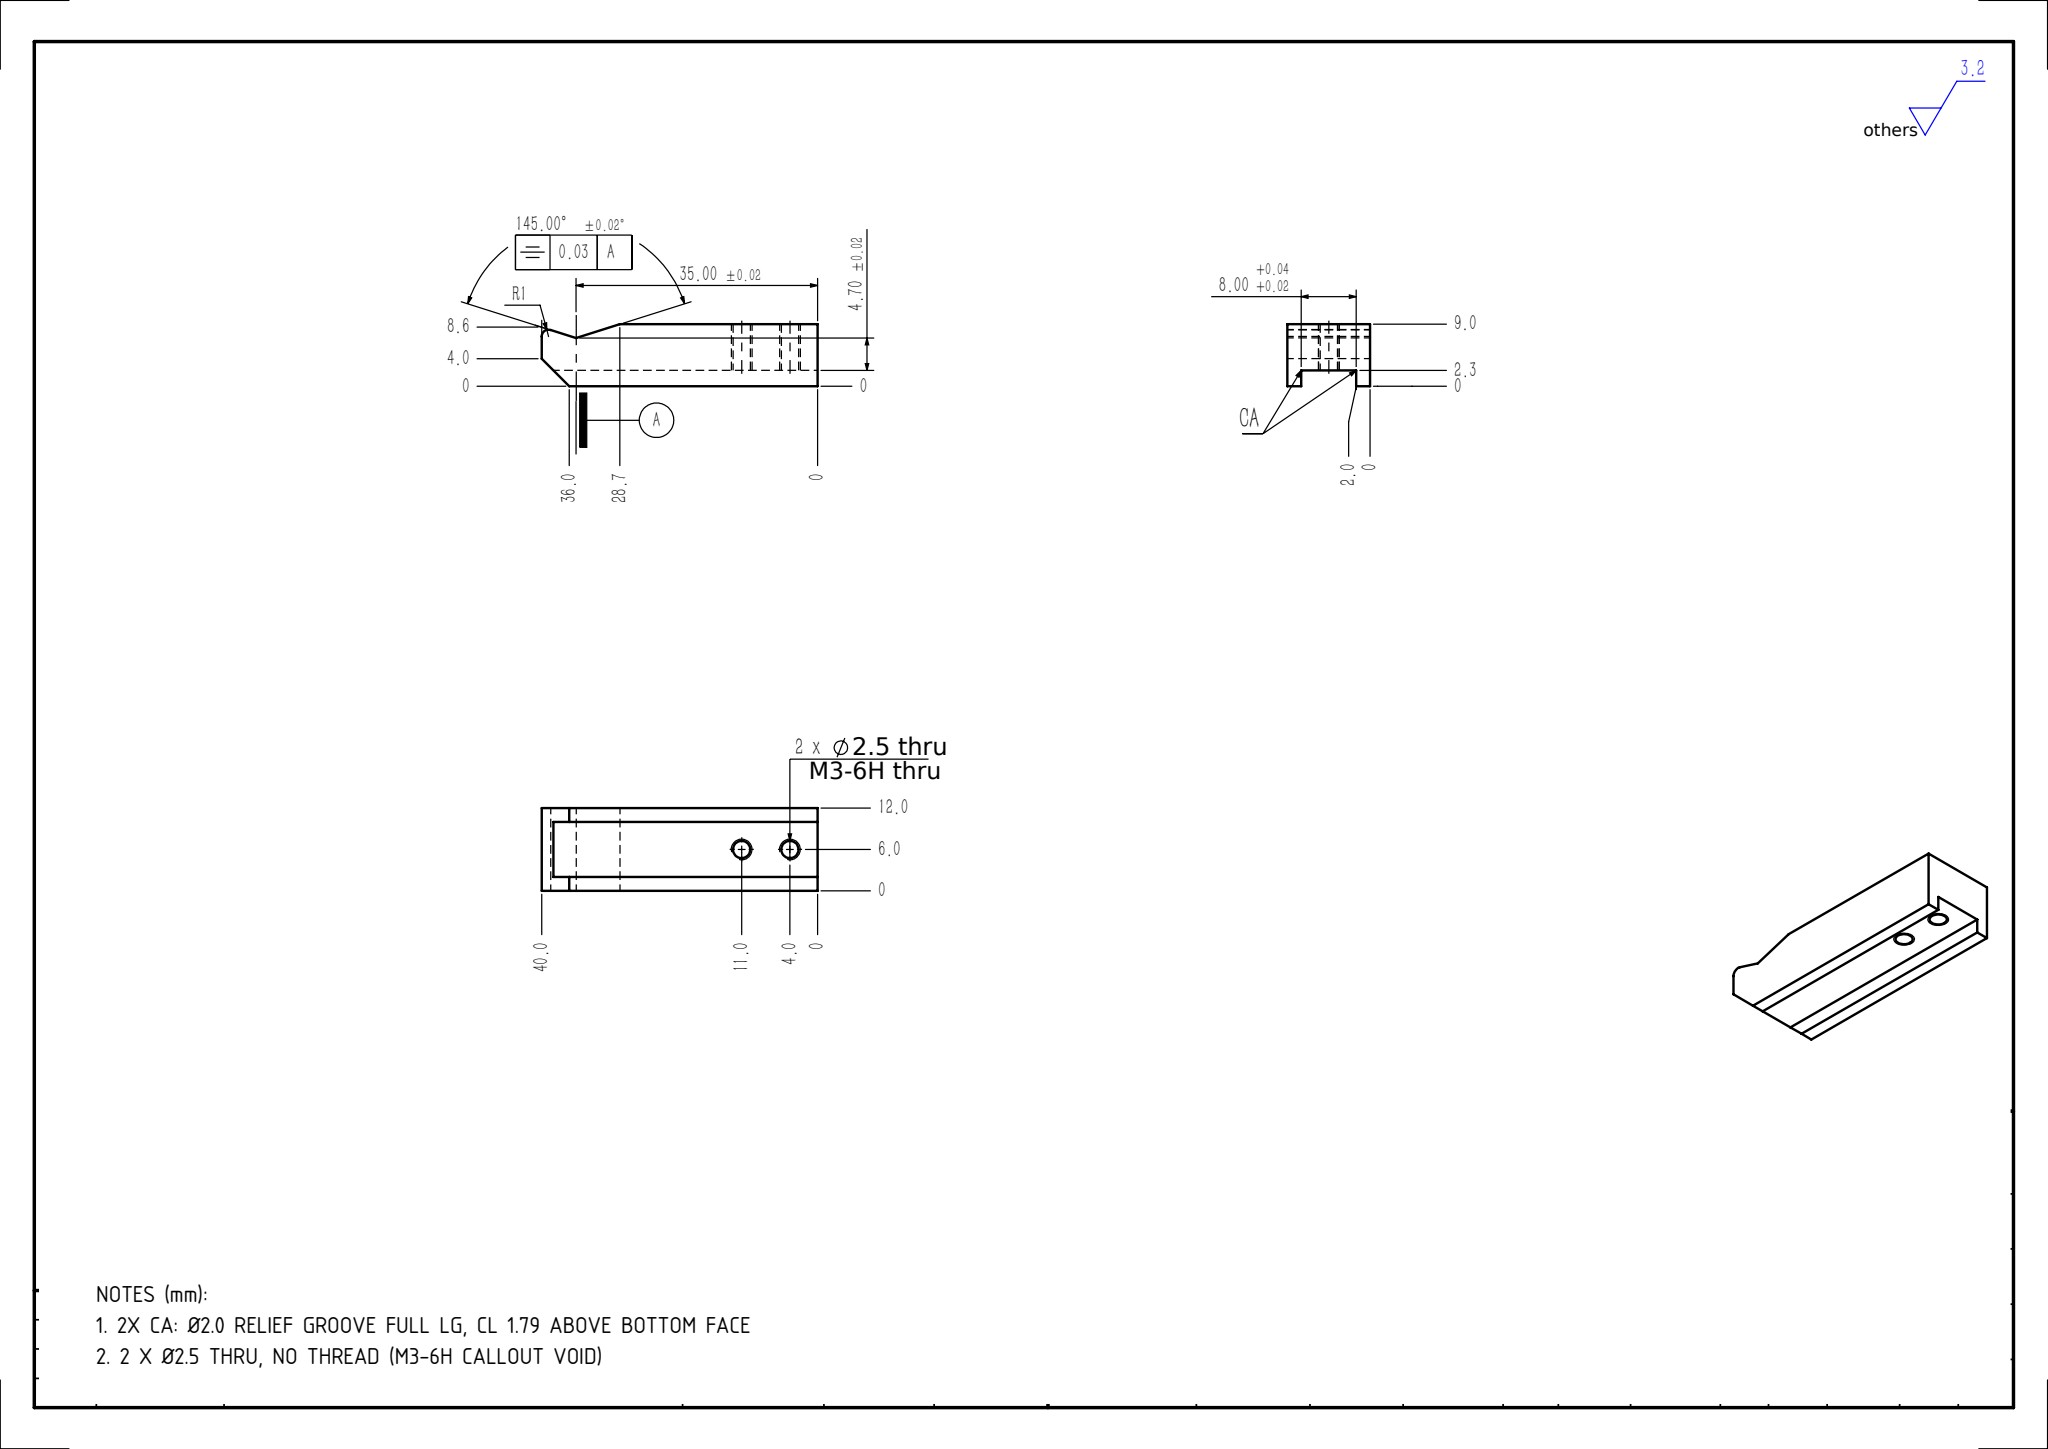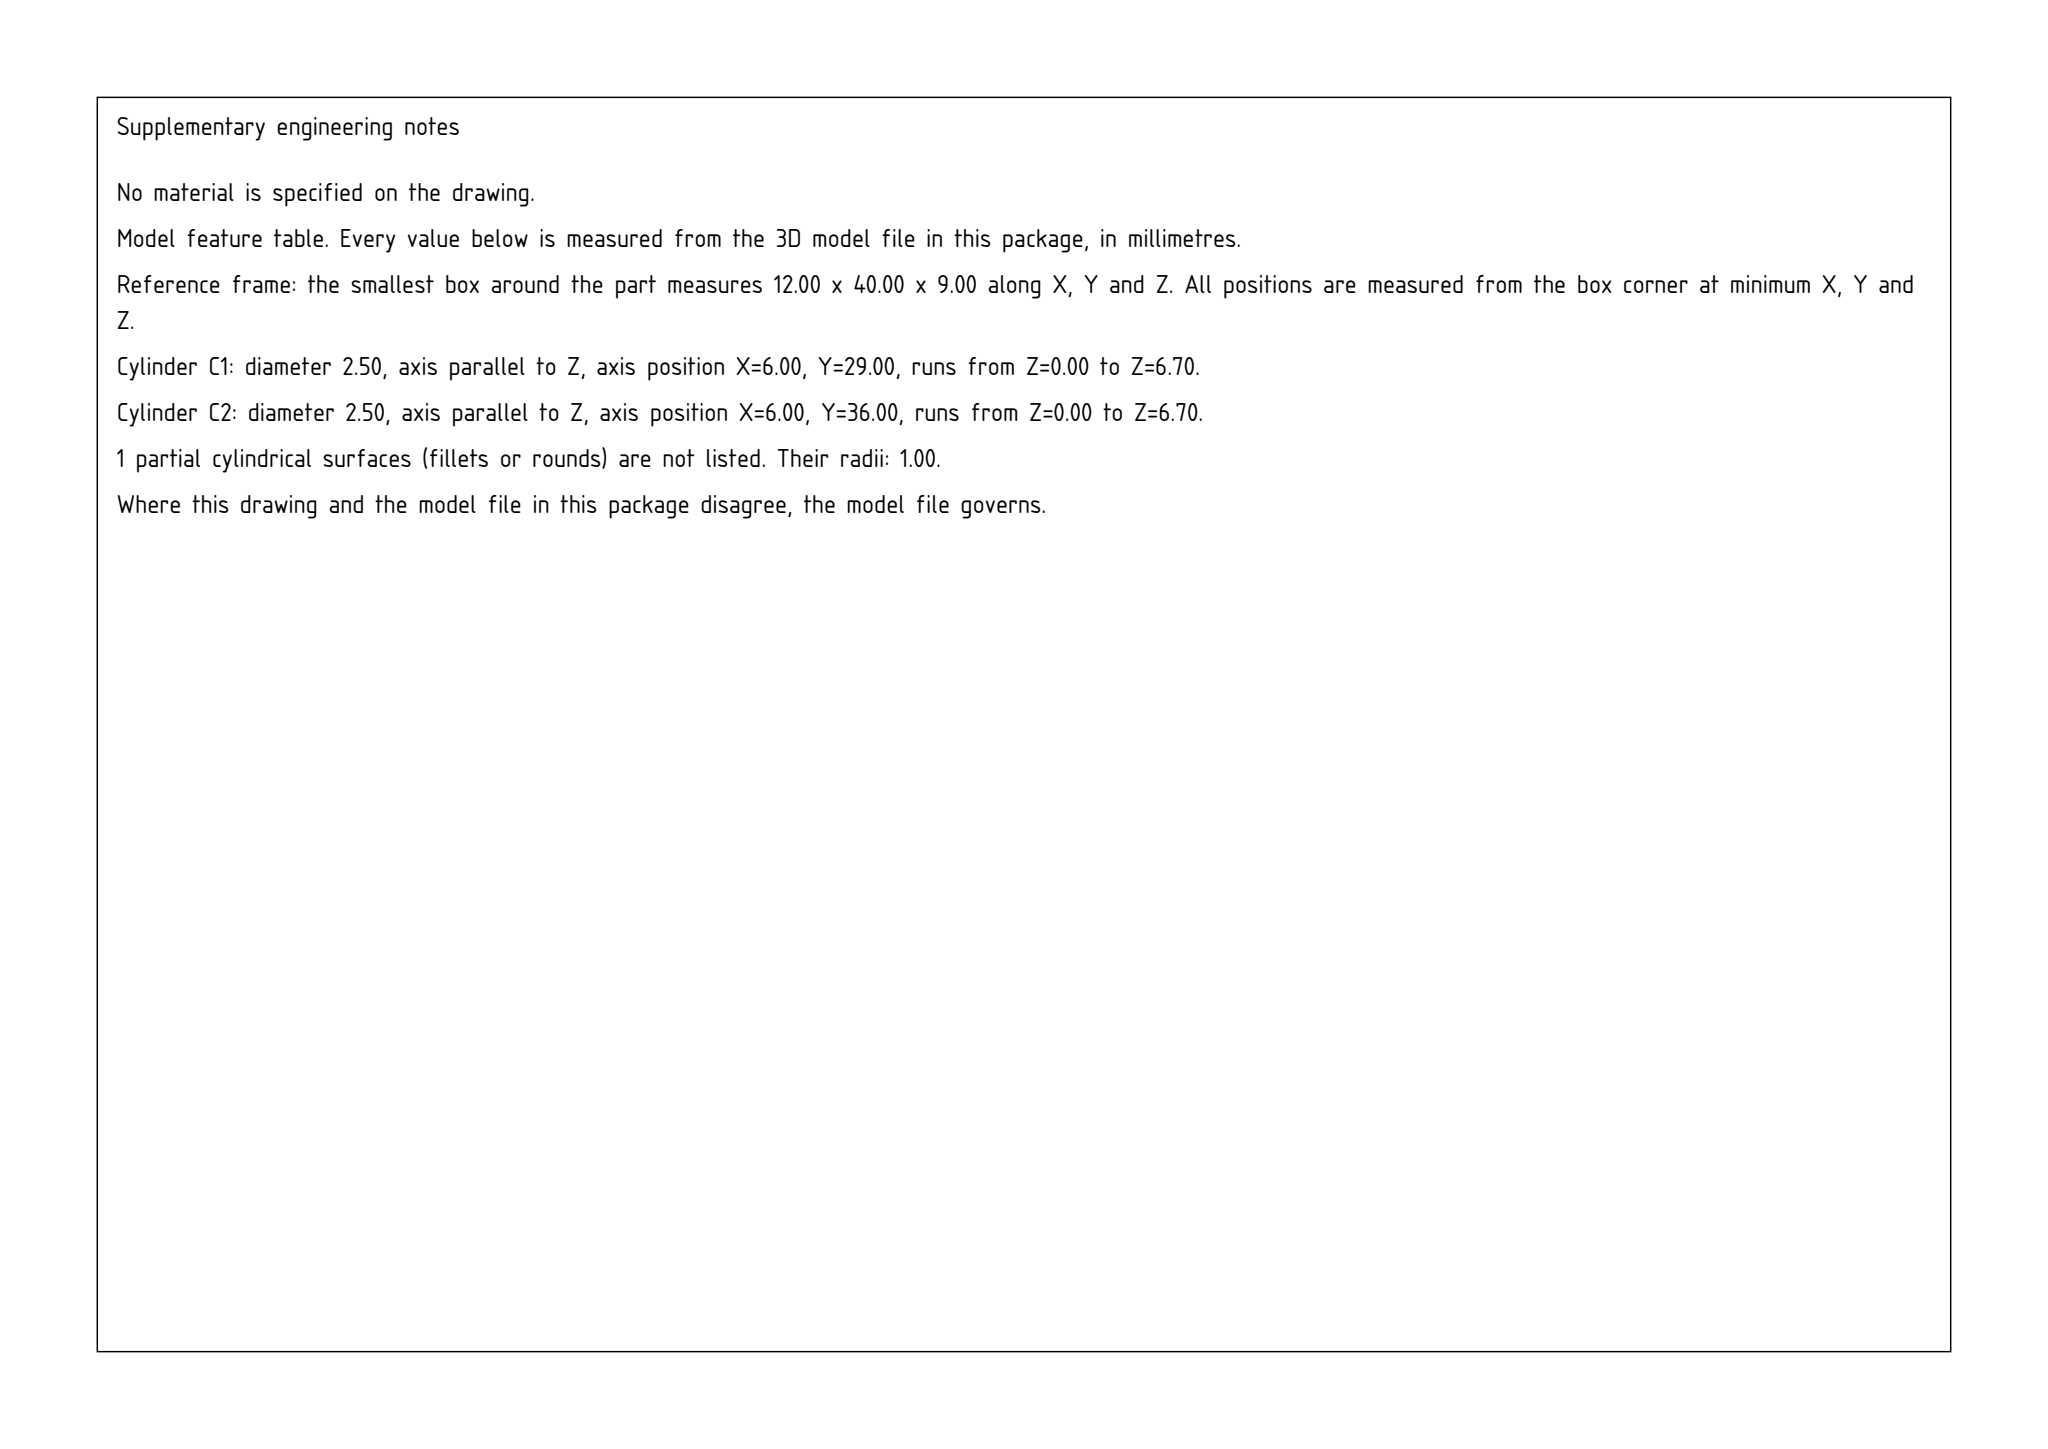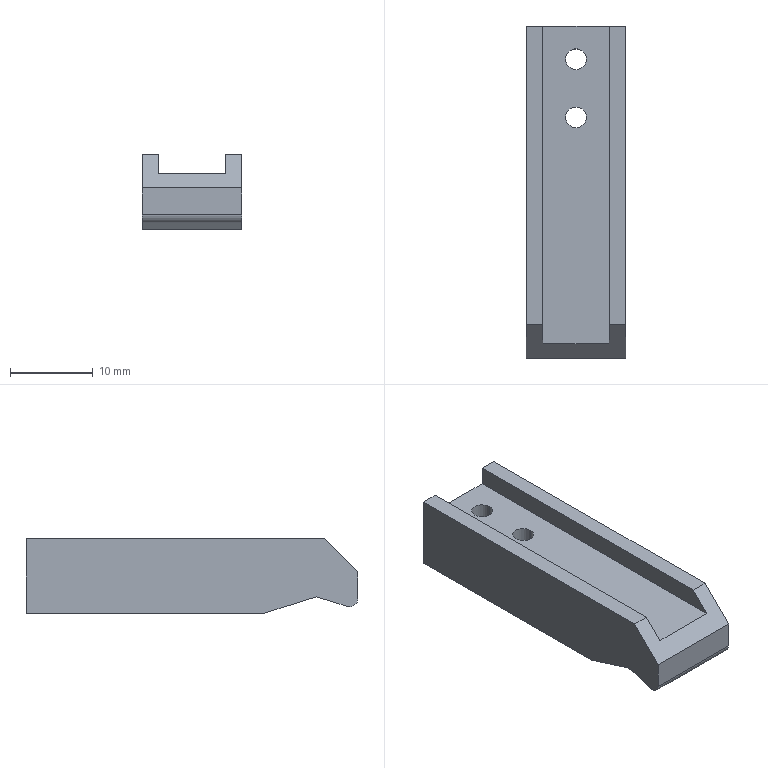Part | SolidWorks | mm | 1 solid | 19 faces | box 12 x 40 x 9 mm | volume 3321 mm3 | plane 13 | cylinder 6 | commonest cylinder face diameters 2.5 x4 2 x2
Drawing notes:
2X CA: Ø2.0 RELIEF GROOVE FULL LG, CL 1.79 ABOVE BOTTOM FACE | from the solid: cylinders [2.0,"x",[null,1.0,1.79],12.0,2] - Ø2.0 grooves, full length, axis 1.79 above z=0 base, at inner corners of 8.00 channel (x=2.0 & x=10.0 walls, floor z=2.3)
2 X Ø2.5 THRU, NO THREAD (M3-6H CALLOUT VOID) | from the solid: cylinders dia 2.5 along z at (x=6.0, y=29.0) and (x=6.0, y=36.0), length 6.7 = full 6.7 wall thickness (z planes 0 and 6.7); no thread/cone features in STEP
STEP:
#1=CARTESIAN_POINT('',(0.,-39.,0.7873));
#2=VERTEX_POINT('',#1);
#3=CARTESIAN_POINT('',(0.,-40.,1.787));
#4=VERTEX_POINT('',#3);
#5=CARTESIAN_POINT('',(0.,-39.,1.787));
#6=DIRECTION('',(-1.,-0.,0.));
#7=DIRECTION('',(-0.,1.,0.));
#8=AXIS2_PLACEMENT_3D('',#5,#6,#7);
#9=CIRCLE('',#8,1.);
#10=EDGE_CURVE('',#2,#4,#9,.T.);
#11=ORIENTED_EDGE('',*,*,#10,.F.);
#12=CARTESIAN_POINT('',(12.,-39.,0.7873));
#13=VERTEX_POINT('',#12);
#14=CARTESIAN_POINT('',(0.,-39.,0.7873));
#15=DIRECTION('',(1.,0.,-0.));
#16=VECTOR('',#15,1000.);
#17=LINE('',#14,#16);
#18=EDGE_CURVE('',#2,#13,#17,.T.);
#19=ORIENTED_EDGE('',*,*,#18,.T.);
#20=CARTESIAN_POINT('',(12.,-40.,1.787));
#21=VERTEX_POINT('',#20);
#22=CARTESIAN_POINT('',(12.,-39.,1.787));
#23=DIRECTION('',(1.,0.,0.));
#24=DIRECTION('',(0.,-1.,0.));
#25=AXIS2_PLACEMENT_3D('',#22,#23,#24);
#26=CIRCLE('',#25,1.);
#27=EDGE_CURVE('',#21,#13,#26,.T.);
#28=ORIENTED_EDGE('',*,*,#27,.F.);
#29=CARTESIAN_POINT('',(0.,-40.,1.787));
#30=DIRECTION('',(1.,0.,-0.));
#31=VECTOR('',#30,1000.);
#32=LINE('',#29,#31);
#33=EDGE_CURVE('',#4,#21,#32,.T.);
#34=ORIENTED_EDGE('',*,*,#33,.F.);
#35=EDGE_LOOP('',(#11,#19,#28,#34));
#36=FACE_OUTER_BOUND('',#35,.T.);
#37=CARTESIAN_POINT('',(0.,-39.,1.787));
#38=DIRECTION('',(1.,0.,-0.));
#39=DIRECTION('',(-0.,0.,-1.));
#40=AXIS2_PLACEMENT_3D('',#37,#38,#39);
#41=CYLINDRICAL_SURFACE('',#40,1.);
#42=ADVANCED_FACE('',(#36),#41,.T.);
#43=CARTESIAN_POINT('',(4.75,-4.,0.));
#44=VERTEX_POINT('',#43);
#45=CARTESIAN_POINT('',(7.25,-4.,0.));
#46=VERTEX_POINT('',#45);
#47=CARTESIAN_POINT('',(6.,-4.,0.));
#48=DIRECTION('',(0.,0.,1.));
#49=DIRECTION('',(1.,0.,0.));
#50=AXIS2_PLACEMENT_3D('',#47,#48,#49);
#51=CIRCLE('',#50,1.25);
#52=EDGE_CURVE('',#44,#46,#51,.T.);
#53=ORIENTED_EDGE('',*,*,#52,.F.);
#54=CARTESIAN_POINT('',(4.75,-4.,6.7));
#55=VERTEX_POINT('',#54);
#56=CARTESIAN_POINT('',(4.75,-4.,6.7));
#57=DIRECTION('',(0.,0.,1.));
#58=VECTOR('',#57,1000.);
#59=LINE('',#56,#58);
#60=EDGE_CURVE('',#44,#55,#59,.T.);
#61=ORIENTED_EDGE('',*,*,#60,.T.);
#62=CARTESIAN_POINT('',(7.25,-4.,6.7));
#63=VERTEX_POINT('',#62);
#64=CARTESIAN_POINT('',(6.,-4.,6.7));
#65=DIRECTION('',(0.,0.,1.));
#66=DIRECTION('',(1.,0.,0.));
#67=AXIS2_PLACEMENT_3D('',#64,#65,#66);
#68=CIRCLE('',#67,1.25);
#69=EDGE_CURVE('',#55,#63,#68,.T.);
#70=ORIENTED_EDGE('',*,*,#69,.T.);
#71=CARTESIAN_POINT('',(7.25,-4.,6.7));
#72=DIRECTION('',(0.,0.,1.));
#73=VECTOR('',#72,1000.);
#74=LINE('',#71,#73);
#75=EDGE_CURVE('',#46,#63,#74,.T.);
#76=ORIENTED_EDGE('',*,*,#75,.F.);
#77=EDGE_LOOP('',(#53,#61,#70,#76));
#78=FACE_OUTER_BOUND('',#77,.T.);
#79=CARTESIAN_POINT('',(6.,-4.,6.7));
#80=DIRECTION('',(0.,0.,1.));
#81=DIRECTION('',(1.,0.,0.));
#82=AXIS2_PLACEMENT_3D('',#79,#80,#81);
#83=CYLINDRICAL_SURFACE('',#82,1.25);
#84=ADVANCED_FACE('',(#78),#83,.F.);
#85=CARTESIAN_POINT('',(4.75,-11.,0.));
#86=VERTEX_POINT('',#85);
#87=CARTESIAN_POINT('',(7.25,-11.,0.));
#88=VERTEX_POINT('',#87);
#89=CARTESIAN_POINT('',(6.,-11.,0.));
#90=DIRECTION('',(0.,0.,1.));
#91=DIRECTION('',(1.,0.,0.));
#92=AXIS2_PLACEMENT_3D('',#89,#90,#91);
#93=CIRCLE('',#92,1.25);
#94=EDGE_CURVE('',#86,#88,#93,.T.);
#95=ORIENTED_EDGE('',*,*,#94,.F.);
#96=CARTESIAN_POINT('',(4.75,-11.,6.7));
#97=VERTEX_POINT('',#96);
#98=CARTESIAN_POINT('',(4.75,-11.,6.7));
#99=DIRECTION('',(0.,0.,1.));
#100=VECTOR('',#99,1000.);
#101=LINE('',#98,#100);
#102=EDGE_CURVE('',#86,#97,#101,.T.);
#103=ORIENTED_EDGE('',*,*,#102,.T.);
#104=CARTESIAN_POINT('',(7.25,-11.,6.7));
#105=VERTEX_POINT('',#104);
#106=CARTESIAN_POINT('',(6.,-11.,6.7));
#107=DIRECTION('',(0.,0.,1.));
#108=DIRECTION('',(1.,0.,0.));
#109=AXIS2_PLACEMENT_3D('',#106,#107,#108);
#110=CIRCLE('',#109,1.25);
#111=EDGE_CURVE('',#97,#105,#110,.T.);
#112=ORIENTED_EDGE('',*,*,#111,.T.);
#113=CARTESIAN_POINT('',(7.25,-11.,6.7));
#114=DIRECTION('',(0.,0.,1.));
#115=VECTOR('',#114,1000.);
#116=LINE('',#113,#115);
#117=EDGE_CURVE('',#88,#105,#116,.T.);
#118=ORIENTED_EDGE('',*,*,#117,.F.);
#119=EDGE_LOOP('',(#95,#103,#112,#118));
#120=FACE_OUTER_BOUND('',#119,.T.);
#121=CARTESIAN_POINT('',(6.,-11.,6.7));
#122=DIRECTION('',(0.,0.,1.));
#123=DIRECTION('',(1.,0.,0.));
#124=AXIS2_PLACEMENT_3D('',#121,#122,#123);
#125=CYLINDRICAL_SURFACE('',#124,1.25);
#126=ADVANCED_FACE('',(#120),#125,.F.);
#127=CARTESIAN_POINT('',(0.,0.,9.));
#128=VERTEX_POINT('',#127);
#129=CARTESIAN_POINT('',(0.,-36.,9.));
#130=VERTEX_POINT('',#129);
#131=CARTESIAN_POINT('',(0.,0.,9.));
#132=DIRECTION('',(0.,-1.,0.));
#133=VECTOR('',#132,1000.);
#134=LINE('',#131,#133);
#135=EDGE_CURVE('',#128,#130,#134,.T.);
#136=ORIENTED_EDGE('',*,*,#135,.T.);
#137=CARTESIAN_POINT('',(2.,-36.,9.));
#138=VERTEX_POINT('',#137);
#139=CARTESIAN_POINT('',(2.,-36.,9.));
#140=DIRECTION('',(1.,0.,0.));
#141=VECTOR('',#140,1000.);
#142=LINE('',#139,#141);
#143=EDGE_CURVE('',#130,#138,#142,.T.);
#144=ORIENTED_EDGE('',*,*,#143,.T.);
#145=CARTESIAN_POINT('',(2.,-0.,9.));
#146=VERTEX_POINT('',#145);
#147=CARTESIAN_POINT('',(2.,-0.,9.));
#148=DIRECTION('',(0.,-1.,0.));
#149=VECTOR('',#148,1000.);
#150=LINE('',#147,#149);
#151=EDGE_CURVE('',#146,#138,#150,.T.);
#152=ORIENTED_EDGE('',*,*,#151,.F.);
#153=CARTESIAN_POINT('',(0.,0.,9.));
#154=DIRECTION('',(-1.,0.,0.));
#155=VECTOR('',#154,1000.);
#156=LINE('',#153,#155);
#157=EDGE_CURVE('',#146,#128,#156,.T.);
#158=ORIENTED_EDGE('',*,*,#157,.T.);
#159=EDGE_LOOP('',(#136,#144,#152,#158));
#160=FACE_OUTER_BOUND('',#159,.T.);
#161=CARTESIAN_POINT('',(0.,0.,9.));
#162=DIRECTION('',(0.,0.,1.));
#163=DIRECTION('',(1.,0.,0.));
#164=AXIS2_PLACEMENT_3D('',#161,#162,#163);
#165=PLANE('',#164);
#166=ADVANCED_FACE('',(#160),#165,.T.);
#167=CARTESIAN_POINT('',(0.,-35.,2.));
#168=VERTEX_POINT('',#167);
#169=CARTESIAN_POINT('',(0.,-38.699,0.8336));
#170=VERTEX_POINT('',#169);
#171=CARTESIAN_POINT('',(0.,-35.,2.));
#172=DIRECTION('',(0.,-0.9537,-0.3007));
#173=VECTOR('',#172,1000.);
#174=LINE('',#171,#173);
#175=EDGE_CURVE('',#168,#170,#174,.T.);
#176=ORIENTED_EDGE('',*,*,#175,.T.);
#177=CARTESIAN_POINT('',(0.,-39.,1.787));
#178=DIRECTION('',(-1.,-0.,0.));
#179=DIRECTION('',(-0.,1.,0.));
#180=AXIS2_PLACEMENT_3D('',#177,#178,#179);
#181=CIRCLE('',#180,1.);
#182=EDGE_CURVE('',#170,#2,#181,.T.);
#183=ORIENTED_EDGE('',*,*,#182,.T.);
#184=ORIENTED_EDGE('',*,*,#10,.T.);
#185=CARTESIAN_POINT('',(0.,-40.,5.));
#186=VERTEX_POINT('',#185);
#187=CARTESIAN_POINT('',(0.,-40.,9.));
#188=DIRECTION('',(0.,0.,-1.));
#189=VECTOR('',#188,1000.);
#190=LINE('',#187,#189);
#191=EDGE_CURVE('',#186,#4,#190,.T.);
#192=ORIENTED_EDGE('',*,*,#191,.F.);
#193=CARTESIAN_POINT('',(0.,-36.,9.));
#194=DIRECTION('',(-0.,0.7071,0.7071));
#195=VECTOR('',#194,1000.);
#196=LINE('',#193,#195);
#197=EDGE_CURVE('',#186,#130,#196,.T.);
#198=ORIENTED_EDGE('',*,*,#197,.T.);
#199=ORIENTED_EDGE('',*,*,#135,.F.);
#200=CARTESIAN_POINT('',(0.,0.,0.));
#201=VERTEX_POINT('',#200);
#202=CARTESIAN_POINT('',(0.,0.,9.));
#203=DIRECTION('',(0.,0.,-1.));
#204=VECTOR('',#203,1000.);
#205=LINE('',#202,#204);
#206=EDGE_CURVE('',#128,#201,#205,.T.);
#207=ORIENTED_EDGE('',*,*,#206,.T.);
#208=CARTESIAN_POINT('',(0.,-28.657,0.));
#209=VERTEX_POINT('',#208);
#210=CARTESIAN_POINT('',(0.,0.,0.));
#211=DIRECTION('',(0.,-1.,0.));
#212=VECTOR('',#211,1000.);
#213=LINE('',#210,#212);
#214=EDGE_CURVE('',#201,#209,#213,.T.);
#215=ORIENTED_EDGE('',*,*,#214,.T.);
#216=CARTESIAN_POINT('',(0.,-28.657,-0.));
#217=DIRECTION('',(0.,-0.9537,0.3007));
#218=VECTOR('',#217,1000.);
#219=LINE('',#216,#218);
#220=EDGE_CURVE('',#209,#168,#219,.T.);
#221=ORIENTED_EDGE('',*,*,#220,.T.);
#222=EDGE_LOOP('',(#176,#183,#184,#192,#198,#199,#207,#215,#221));
#223=FACE_OUTER_BOUND('',#222,.T.);
#224=CARTESIAN_POINT('',(0.,0.,9.));
#225=DIRECTION('',(1.,0.,0.));
#226=DIRECTION('',(-0.,1.,0.));
#227=AXIS2_PLACEMENT_3D('',#224,#225,#226);
#228=PLANE('',#227);
#229=ADVANCED_FACE('',(#223),#228,.F.);
#230=ORIENTED_EDGE('',*,*,#191,.T.);
#231=ORIENTED_EDGE('',*,*,#33,.T.);
#232=CARTESIAN_POINT('',(12.,-40.,5.));
#233=VERTEX_POINT('',#232);
#234=CARTESIAN_POINT('',(12.,-40.,9.));
#235=DIRECTION('',(0.,0.,-1.));
#236=VECTOR('',#235,1000.);
#237=LINE('',#234,#236);
#238=EDGE_CURVE('',#233,#21,#237,.T.);
#239=ORIENTED_EDGE('',*,*,#238,.F.);
#240=CARTESIAN_POINT('',(10.,-40.,5.));
#241=DIRECTION('',(-1.,0.,0.));
#242=VECTOR('',#241,1000.);
#243=LINE('',#240,#242);
#244=EDGE_CURVE('',#233,#186,#243,.T.);
#245=ORIENTED_EDGE('',*,*,#244,.T.);
#246=EDGE_LOOP('',(#230,#231,#239,#245));
#247=FACE_OUTER_BOUND('',#246,.T.);
#248=CARTESIAN_POINT('',(0.,-40.,9.));
#249=DIRECTION('',(0.,1.,0.));
#250=DIRECTION('',(0.,0.,1.));
#251=AXIS2_PLACEMENT_3D('',#248,#249,#250);
#252=PLANE('',#251);
#253=ADVANCED_FACE('',(#247),#252,.F.);
#254=ORIENTED_EDGE('',*,*,#238,.T.);
#255=ORIENTED_EDGE('',*,*,#27,.T.);
#256=CARTESIAN_POINT('',(12.,-38.699,0.8336));
#257=VERTEX_POINT('',#256);
#258=CARTESIAN_POINT('',(12.,-39.,1.787));
#259=DIRECTION('',(1.,0.,0.));
#260=DIRECTION('',(0.,-1.,0.));
#261=AXIS2_PLACEMENT_3D('',#258,#259,#260);
#262=CIRCLE('',#261,1.);
#263=EDGE_CURVE('',#13,#257,#262,.T.);
#264=ORIENTED_EDGE('',*,*,#263,.T.);
#265=CARTESIAN_POINT('',(12.,-35.,2.));
#266=VERTEX_POINT('',#265);
#267=CARTESIAN_POINT('',(12.,-35.,2.));
#268=DIRECTION('',(0.,-0.9537,-0.3007));
#269=VECTOR('',#268,1000.);
#270=LINE('',#267,#269);
#271=EDGE_CURVE('',#266,#257,#270,.T.);
#272=ORIENTED_EDGE('',*,*,#271,.F.);
#273=CARTESIAN_POINT('',(12.,-28.657,-0.));
#274=VERTEX_POINT('',#273);
#275=CARTESIAN_POINT('',(12.,-28.657,-0.));
#276=DIRECTION('',(0.,-0.9537,0.3007));
#277=VECTOR('',#276,1000.);
#278=LINE('',#275,#277);
#279=EDGE_CURVE('',#274,#266,#278,.T.);
#280=ORIENTED_EDGE('',*,*,#279,.F.);
#281=CARTESIAN_POINT('',(12.,0.,0.));
#282=VERTEX_POINT('',#281);
#283=CARTESIAN_POINT('',(12.,0.,0.));
#284=DIRECTION('',(-0.,1.,0.));
#285=VECTOR('',#284,1000.);
#286=LINE('',#283,#285);
#287=EDGE_CURVE('',#274,#282,#286,.T.);
#288=ORIENTED_EDGE('',*,*,#287,.T.);
#289=CARTESIAN_POINT('',(12.,0.,9.));
#290=VERTEX_POINT('',#289);
#291=CARTESIAN_POINT('',(12.,0.,9.));
#292=DIRECTION('',(0.,0.,-1.));
#293=VECTOR('',#292,1000.);
#294=LINE('',#291,#293);
#295=EDGE_CURVE('',#290,#282,#294,.T.);
#296=ORIENTED_EDGE('',*,*,#295,.F.);
#297=CARTESIAN_POINT('',(12.,-36.,9.));
#298=VERTEX_POINT('',#297);
#299=CARTESIAN_POINT('',(12.,0.,9.));
#300=DIRECTION('',(-0.,1.,0.));
#301=VECTOR('',#300,1000.);
#302=LINE('',#299,#301);
#303=EDGE_CURVE('',#298,#290,#302,.T.);
#304=ORIENTED_EDGE('',*,*,#303,.F.);
#305=CARTESIAN_POINT('',(12.,-36.,9.));
#306=DIRECTION('',(0.,-0.7071,-0.7071));
#307=VECTOR('',#306,1000.);
#308=LINE('',#305,#307);
#309=EDGE_CURVE('',#298,#233,#308,.T.);
#310=ORIENTED_EDGE('',*,*,#309,.T.);
#311=EDGE_LOOP('',(#254,#255,#264,#272,#280,#288,#296,#304,#310));
#312=FACE_OUTER_BOUND('',#311,.T.);
#313=CARTESIAN_POINT('',(12.,0.,9.));
#314=DIRECTION('',(-1.,-0.,0.));
#315=DIRECTION('',(0.,-1.,0.));
#316=AXIS2_PLACEMENT_3D('',#313,#314,#315);
#317=PLANE('',#316);
#318=ADVANCED_FACE('',(#312),#317,.F.);
#319=ORIENTED_EDGE('',*,*,#157,.F.);
#320=CARTESIAN_POINT('',(2.,-0.,6.7));
#321=VERTEX_POINT('',#320);
#322=CARTESIAN_POINT('',(2.,-0.,6.7));
#323=DIRECTION('',(0.,0.,1.));
#324=VECTOR('',#323,1000.);
#325=LINE('',#322,#324);
#326=EDGE_CURVE('',#321,#146,#325,.T.);
#327=ORIENTED_EDGE('',*,*,#326,.F.);
#328=CARTESIAN_POINT('',(10.,-0.,6.7));
#329=VERTEX_POINT('',#328);
#330=CARTESIAN_POINT('',(2.,-0.,6.7));
#331=DIRECTION('',(-1.,-0.,0.));
#332=VECTOR('',#331,1000.);
#333=LINE('',#330,#332);
#334=EDGE_CURVE('',#329,#321,#333,.T.);
#335=ORIENTED_EDGE('',*,*,#334,.F.);
#336=CARTESIAN_POINT('',(10.,-0.,9.));
#337=VERTEX_POINT('',#336);
#338=CARTESIAN_POINT('',(10.,-0.,6.7));
#339=DIRECTION('',(0.,0.,1.));
#340=VECTOR('',#339,1000.);
#341=LINE('',#338,#340);
#342=EDGE_CURVE('',#329,#337,#341,.T.);
#343=ORIENTED_EDGE('',*,*,#342,.T.);
#344=CARTESIAN_POINT('',(0.,0.,9.));
#345=DIRECTION('',(-1.,0.,0.));
#346=VECTOR('',#345,1000.);
#347=LINE('',#344,#346);
#348=EDGE_CURVE('',#290,#337,#347,.T.);
#349=ORIENTED_EDGE('',*,*,#348,.F.);
#350=ORIENTED_EDGE('',*,*,#295,.T.);
#351=CARTESIAN_POINT('',(0.,0.,0.));
#352=DIRECTION('',(-1.,0.,0.));
#353=VECTOR('',#352,1000.);
#354=LINE('',#351,#353);
#355=EDGE_CURVE('',#282,#201,#354,.T.);
#356=ORIENTED_EDGE('',*,*,#355,.T.);
#357=ORIENTED_EDGE('',*,*,#206,.F.);
#358=EDGE_LOOP('',(#319,#327,#335,#343,#349,#350,#356,#357));
#359=FACE_OUTER_BOUND('',#358,.T.);
#360=CARTESIAN_POINT('',(0.,0.,9.));
#361=DIRECTION('',(0.,-1.,0.));
#362=DIRECTION('',(0.,0.,-1.));
#363=AXIS2_PLACEMENT_3D('',#360,#361,#362);
#364=PLANE('',#363);
#365=ADVANCED_FACE('',(#359),#364,.F.);
#366=CARTESIAN_POINT('',(10.,-36.,9.));
#367=VERTEX_POINT('',#366);
#368=CARTESIAN_POINT('',(10.,-0.,9.));
#369=DIRECTION('',(-0.,1.,0.));
#370=VECTOR('',#369,1000.);
#371=LINE('',#368,#370);
#372=EDGE_CURVE('',#367,#337,#371,.T.);
#373=ORIENTED_EDGE('',*,*,#372,.F.);
#374=CARTESIAN_POINT('',(12.,-36.,9.));
#375=DIRECTION('',(1.,0.,0.));
#376=VECTOR('',#375,1000.);
#377=LINE('',#374,#376);
#378=EDGE_CURVE('',#367,#298,#377,.T.);
#379=ORIENTED_EDGE('',*,*,#378,.T.);
#380=ORIENTED_EDGE('',*,*,#303,.T.);
#381=ORIENTED_EDGE('',*,*,#348,.T.);
#382=EDGE_LOOP('',(#373,#379,#380,#381));
#383=FACE_OUTER_BOUND('',#382,.T.);
#384=CARTESIAN_POINT('',(0.,0.,9.));
#385=DIRECTION('',(0.,0.,1.));
#386=DIRECTION('',(1.,0.,0.));
#387=AXIS2_PLACEMENT_3D('',#384,#385,#386);
#388=PLANE('',#387);
#389=ADVANCED_FACE('',(#383),#388,.T.);
#390=CARTESIAN_POINT('',(6.,-4.,0.));
#391=DIRECTION('',(0.,0.,1.));
#392=DIRECTION('',(1.,0.,0.));
#393=AXIS2_PLACEMENT_3D('',#390,#391,#392);
#394=CIRCLE('',#393,1.25);
#395=EDGE_CURVE('',#46,#44,#394,.T.);
#396=ORIENTED_EDGE('',*,*,#395,.T.);
#397=ORIENTED_EDGE('',*,*,#52,.T.);
#398=EDGE_LOOP('',(#396,#397));
#399=FACE_BOUND('',#398,.T.);
#400=CARTESIAN_POINT('',(6.,-11.,0.));
#401=DIRECTION('',(0.,0.,1.));
#402=DIRECTION('',(1.,0.,0.));
#403=AXIS2_PLACEMENT_3D('',#400,#401,#402);
#404=CIRCLE('',#403,1.25);
#405=EDGE_CURVE('',#88,#86,#404,.T.);
#406=ORIENTED_EDGE('',*,*,#405,.T.);
#407=ORIENTED_EDGE('',*,*,#94,.T.);
#408=EDGE_LOOP('',(#406,#407));
#409=FACE_BOUND('',#408,.T.);
#410=ORIENTED_EDGE('',*,*,#287,.F.);
#411=CARTESIAN_POINT('',(0.,-28.657,-0.));
#412=DIRECTION('',(1.,0.,0.));
#413=VECTOR('',#412,1000.);
#414=LINE('',#411,#413);
#415=EDGE_CURVE('',#209,#274,#414,.T.);
#416=ORIENTED_EDGE('',*,*,#415,.F.);
#417=ORIENTED_EDGE('',*,*,#214,.F.);
#418=ORIENTED_EDGE('',*,*,#355,.F.);
#419=EDGE_LOOP('',(#410,#416,#417,#418));
#420=FACE_OUTER_BOUND('',#419,.T.);
#421=CARTESIAN_POINT('',(0.,0.,0.));
#422=DIRECTION('',(0.,0.,1.));
#423=DIRECTION('',(1.,0.,0.));
#424=AXIS2_PLACEMENT_3D('',#421,#422,#423);
#425=PLANE('',#424);
#426=ADVANCED_FACE('',(#399,#409,#420),#425,.F.);
#427=ORIENTED_EDGE('',*,*,#271,.T.);
#428=CARTESIAN_POINT('',(-0.,-38.699,0.8336));
#429=DIRECTION('',(-1.,0.,0.));
#430=VECTOR('',#429,1000.);
#431=LINE('',#428,#430);
#432=EDGE_CURVE('',#257,#170,#431,.T.);
#433=ORIENTED_EDGE('',*,*,#432,.T.);
#434=ORIENTED_EDGE('',*,*,#175,.F.);
#435=CARTESIAN_POINT('',(0.,-35.,2.));
#436=DIRECTION('',(1.,0.,0.));
#437=VECTOR('',#436,1000.);
#438=LINE('',#435,#437);
#439=EDGE_CURVE('',#168,#266,#438,.T.);
#440=ORIENTED_EDGE('',*,*,#439,.T.);
#441=EDGE_LOOP('',(#427,#433,#434,#440));
#442=FACE_OUTER_BOUND('',#441,.T.);
#443=CARTESIAN_POINT('',(0.,-35.,2.));
#444=DIRECTION('',(0.,-0.3007,0.9537));
#445=DIRECTION('',(0.,-0.9537,-0.3007));
#446=AXIS2_PLACEMENT_3D('',#443,#444,#445);
#447=PLANE('',#446);
#448=ADVANCED_FACE('',(#442),#447,.F.);
#449=ORIENTED_EDGE('',*,*,#279,.T.);
#450=ORIENTED_EDGE('',*,*,#439,.F.);
#451=ORIENTED_EDGE('',*,*,#220,.F.);
#452=ORIENTED_EDGE('',*,*,#415,.T.);
#453=EDGE_LOOP('',(#449,#450,#451,#452));
#454=FACE_OUTER_BOUND('',#453,.T.);
#455=CARTESIAN_POINT('',(0.,-28.657,-0.));
#456=DIRECTION('',(-0.,0.3007,0.9537));
#457=DIRECTION('',(0.,-0.9537,0.3007));
#458=AXIS2_PLACEMENT_3D('',#455,#456,#457);
#459=PLANE('',#458);
#460=ADVANCED_FACE('',(#454),#459,.F.);
#461=ORIENTED_EDGE('',*,*,#151,.T.);
#462=CARTESIAN_POINT('',(2.,-38.3,6.7));
#463=VERTEX_POINT('',#462);
#464=CARTESIAN_POINT('',(2.,-36.,9.));
#465=DIRECTION('',(0.,-0.7071,-0.7071));
#466=VECTOR('',#465,1000.);
#467=LINE('',#464,#466);
#468=EDGE_CURVE('',#138,#463,#467,.T.);
#469=ORIENTED_EDGE('',*,*,#468,.T.);
#470=CARTESIAN_POINT('',(2.,-0.,6.7));
#471=DIRECTION('',(0.,-1.,0.));
#472=VECTOR('',#471,1000.);
#473=LINE('',#470,#472);
#474=EDGE_CURVE('',#321,#463,#473,.T.);
#475=ORIENTED_EDGE('',*,*,#474,.F.);
#476=ORIENTED_EDGE('',*,*,#326,.T.);
#477=EDGE_LOOP('',(#461,#469,#475,#476));
#478=FACE_OUTER_BOUND('',#477,.T.);
#479=CARTESIAN_POINT('',(2.,-0.,6.7));
#480=DIRECTION('',(-1.,-0.,0.));
#481=DIRECTION('',(0.,-1.,0.));
#482=AXIS2_PLACEMENT_3D('',#479,#480,#481);
#483=PLANE('',#482);
#484=ADVANCED_FACE('',(#478),#483,.F.);
#485=CARTESIAN_POINT('',(10.,-38.3,6.7));
#486=VERTEX_POINT('',#485);
#487=CARTESIAN_POINT('',(10.,-0.,6.7));
#488=DIRECTION('',(-0.,1.,0.));
#489=VECTOR('',#488,1000.);
#490=LINE('',#487,#489);
#491=EDGE_CURVE('',#486,#329,#490,.T.);
#492=ORIENTED_EDGE('',*,*,#491,.F.);
#493=CARTESIAN_POINT('',(10.,-36.,9.));
#494=DIRECTION('',(-0.,0.7071,0.7071));
#495=VECTOR('',#494,1000.);
#496=LINE('',#493,#495);
#497=EDGE_CURVE('',#486,#367,#496,.T.);
#498=ORIENTED_EDGE('',*,*,#497,.T.);
#499=ORIENTED_EDGE('',*,*,#372,.T.);
#500=ORIENTED_EDGE('',*,*,#342,.F.);
#501=EDGE_LOOP('',(#492,#498,#499,#500));
#502=FACE_OUTER_BOUND('',#501,.T.);
#503=CARTESIAN_POINT('',(10.,-0.,6.7));
#504=DIRECTION('',(1.,0.,0.));
#505=DIRECTION('',(-0.,1.,0.));
#506=AXIS2_PLACEMENT_3D('',#503,#504,#505);
#507=PLANE('',#506);
#508=ADVANCED_FACE('',(#502),#507,.F.);
#509=CARTESIAN_POINT('',(6.,-4.,6.7));
#510=DIRECTION('',(0.,0.,1.));
#511=DIRECTION('',(1.,0.,0.));
#512=AXIS2_PLACEMENT_3D('',#509,#510,#511);
#513=CIRCLE('',#512,1.25);
#514=EDGE_CURVE('',#63,#55,#513,.T.);
#515=ORIENTED_EDGE('',*,*,#514,.F.);
#516=ORIENTED_EDGE('',*,*,#69,.F.);
#517=EDGE_LOOP('',(#515,#516));
#518=FACE_BOUND('',#517,.T.);
#519=CARTESIAN_POINT('',(6.,-11.,6.7));
#520=DIRECTION('',(0.,0.,1.));
#521=DIRECTION('',(1.,0.,0.));
#522=AXIS2_PLACEMENT_3D('',#519,#520,#521);
#523=CIRCLE('',#522,1.25);
#524=EDGE_CURVE('',#105,#97,#523,.T.);
#525=ORIENTED_EDGE('',*,*,#524,.F.);
#526=ORIENTED_EDGE('',*,*,#111,.F.);
#527=EDGE_LOOP('',(#525,#526));
#528=FACE_BOUND('',#527,.T.);
#529=ORIENTED_EDGE('',*,*,#474,.T.);
#530=CARTESIAN_POINT('',(0.,-38.3,6.7));
#531=DIRECTION('',(1.,0.,0.));
#532=VECTOR('',#531,1000.);
#533=LINE('',#530,#532);
#534=EDGE_CURVE('',#463,#486,#533,.T.);
#535=ORIENTED_EDGE('',*,*,#534,.T.);
#536=ORIENTED_EDGE('',*,*,#491,.T.);
#537=ORIENTED_EDGE('',*,*,#334,.T.);
#538=EDGE_LOOP('',(#529,#535,#536,#537));
#539=FACE_OUTER_BOUND('',#538,.T.);
#540=CARTESIAN_POINT('',(0.,0.,6.7));
#541=DIRECTION('',(0.,0.,1.));
#542=DIRECTION('',(1.,0.,0.));
#543=AXIS2_PLACEMENT_3D('',#540,#541,#542);
#544=PLANE('',#543);
#545=ADVANCED_FACE('',(#518,#528,#539),#544,.T.);
#546=ORIENTED_EDGE('',*,*,#102,.F.);
#547=ORIENTED_EDGE('',*,*,#405,.F.);
#548=ORIENTED_EDGE('',*,*,#117,.T.);
#549=ORIENTED_EDGE('',*,*,#524,.T.);
#550=EDGE_LOOP('',(#546,#547,#548,#549));
#551=FACE_OUTER_BOUND('',#550,.T.);
#552=CARTESIAN_POINT('',(6.,-11.,6.7));
#553=DIRECTION('',(0.,0.,1.));
#554=DIRECTION('',(1.,0.,0.));
#555=AXIS2_PLACEMENT_3D('',#552,#553,#554);
#556=CYLINDRICAL_SURFACE('',#555,1.25);
#557=ADVANCED_FACE('',(#551),#556,.F.);
#558=ORIENTED_EDGE('',*,*,#60,.F.);
#559=ORIENTED_EDGE('',*,*,#395,.F.);
#560=ORIENTED_EDGE('',*,*,#75,.T.);
#561=ORIENTED_EDGE('',*,*,#514,.T.);
#562=EDGE_LOOP('',(#558,#559,#560,#561));
#563=FACE_OUTER_BOUND('',#562,.T.);
#564=CARTESIAN_POINT('',(6.,-4.,6.7));
#565=DIRECTION('',(0.,0.,1.));
#566=DIRECTION('',(1.,0.,0.));
#567=AXIS2_PLACEMENT_3D('',#564,#565,#566);
#568=CYLINDRICAL_SURFACE('',#567,1.25);
#569=ADVANCED_FACE('',(#563),#568,.F.);
#570=ORIENTED_EDGE('',*,*,#497,.F.);
#571=ORIENTED_EDGE('',*,*,#534,.F.);
#572=ORIENTED_EDGE('',*,*,#468,.F.);
#573=ORIENTED_EDGE('',*,*,#143,.F.);
#574=ORIENTED_EDGE('',*,*,#197,.F.);
#575=ORIENTED_EDGE('',*,*,#244,.F.);
#576=ORIENTED_EDGE('',*,*,#309,.F.);
#577=ORIENTED_EDGE('',*,*,#378,.F.);
#578=EDGE_LOOP('',(#570,#571,#572,#573,#574,#575,#576,#577));
#579=FACE_OUTER_BOUND('',#578,.T.);
#580=CARTESIAN_POINT('',(0.,-36.,9.));
#581=DIRECTION('',(0.,-0.7071,0.7071));
#582=DIRECTION('',(-1.,0.,0.));
#583=AXIS2_PLACEMENT_3D('',#580,#581,#582);
#584=PLANE('',#583);
#585=ADVANCED_FACE('',(#579),#584,.T.);
#586=ORIENTED_EDGE('',*,*,#18,.F.);
#587=ORIENTED_EDGE('',*,*,#182,.F.);
#588=ORIENTED_EDGE('',*,*,#432,.F.);
#589=ORIENTED_EDGE('',*,*,#263,.F.);
#590=EDGE_LOOP('',(#586,#587,#588,#589));
#591=FACE_OUTER_BOUND('',#590,.T.);
#592=CARTESIAN_POINT('',(0.,-39.,1.787));
#593=DIRECTION('',(1.,0.,-0.));
#594=DIRECTION('',(-0.,0.,-1.));
#595=AXIS2_PLACEMENT_3D('',#592,#593,#594);
#596=CYLINDRICAL_SURFACE('',#595,1.);
#597=ADVANCED_FACE('',(#591),#596,.T.);
#598=CLOSED_SHELL('',(#42,#84,#126,#166,#229,#253,#318,#365,#389,#426,#448,#460,#484,#508,#545,#557,#569,#585,#597));
#599=MANIFOLD_SOLID_BREP('',#598);
#600=CARTESIAN_POINT('',(0.,0.,0.));
#601=DIRECTION('',(0.,0.,1.));
#602=DIRECTION('',(1.,0.,0.));
#603=AXIS2_PLACEMENT_3D('',#600,#601,#602);
#604=(LENGTH_UNIT()NAMED_UNIT(*)SI_UNIT(.MILLI.,.METRE.));
#605=UNCERTAINTY_MEASURE_WITH_UNIT(LENGTH_MEASURE(0.00001),#604,'','');
#606=(NAMED_UNIT(*)PLANE_ANGLE_UNIT()SI_UNIT($,.RADIAN.));
#607=(NAMED_UNIT(*)SI_UNIT($,.STERADIAN.)SOLID_ANGLE_UNIT());
#608=(GEOMETRIC_REPRESENTATION_CONTEXT(3)GLOBAL_UNCERTAINTY_ASSIGNED_CONTEXT((#605))GLOBAL_UNIT_ASSIGNED_CONTEXT((#604,#606,#607))REPRESENTATION_CONTEXT('',''));
#609=ADVANCED_BREP_SHAPE_REPRESENTATION('',(#599,#603),#608);